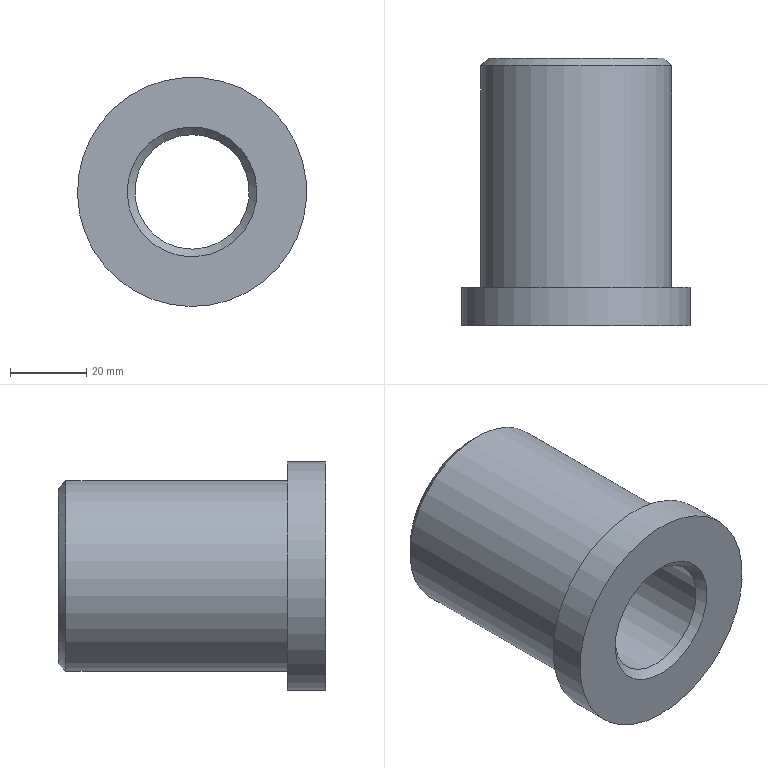Component | NX | SPINDLE_SLEEVE | 1 solid | 9 faces | box 60 x 70 x 60 mm | volume 95904 mm3 | plane 3 | cylinder 3 | cone 3 | commonest cylinder face diameters 30 x1 60 x1 50 x1
STEP:
#1=CARTESIAN_POINT('',(0.,0.,0.));
#2=DIRECTION('',(0.,0.,1.));
#3=DIRECTION('',(1.,0.,0.));
#4=AXIS2_PLACEMENT_3D('',#1,#2,#3);
#5=CARTESIAN_POINT('',(289.146,-15.,110.278));
#6=VERTEX_POINT('',#5);
#7=CARTESIAN_POINT('',(300.,-15.,90.));
#8=DIRECTION('',(0.,1.,0.));
#9=DIRECTION('',(-0.4719,0.,0.8817));
#10=AXIS2_PLACEMENT_3D('',#7,#8,#9);
#11=CIRCLE('',#10,23.);
#12=CARTESIAN_POINT('',(322.041,-15.,101.797));
#13=DIRECTION('',(0.,1.,0.));
#14=DIRECTION('',(-0.4719,0.,0.8817));
#15=AXIS2_PLACEMENT_3D('',#12,#13,#14);
#16=PLANE('',#15);
#17=CARTESIAN_POINT('',(-0.,-25.));
#18=DIRECTION('',(1.,0.));
#19=AXIS2_PLACEMENT_2D('',#17,#18);
#20=CIRCLE('',#19,23.);
#21=(GEOMETRIC_REPRESENTATION_CONTEXT(2)PARAMETRIC_REPRESENTATION_CONTEXT()REPRESENTATION_CONTEXT('',''));
#22=DEFINITIONAL_REPRESENTATION('',(#20),#21);
#23=PCURVE('',#16,#22);
#24=CARTESIAN_POINT('',(300.,-17.,90.));
#25=DIRECTION('',(0.,-1.,0.));
#26=DIRECTION('',(0.4719,0.,-0.8817));
#27=AXIS2_PLACEMENT_3D('',#24,#25,#26);
#28=CONICAL_SURFACE('',#27,25.,0.7854);
#29=CARTESIAN_POINT('',(9.425,-2.));
#30=DIRECTION('',(-1.,0.));
#31=VECTOR('',#30,1.);
#32=LINE('',#29,#31);
#33=(GEOMETRIC_REPRESENTATION_CONTEXT(2)PARAMETRIC_REPRESENTATION_CONTEXT()REPRESENTATION_CONTEXT('',''));
#34=DEFINITIONAL_REPRESENTATION('',(#32),#33);
#35=PCURVE('',#28,#34);
#36=SURFACE_CURVE('',#11,(#23,#35),.PCURVE_S1.);
#37=EDGE_CURVE('',#6,#6,#36,.T.);
#38=ORIENTED_EDGE('',*,*,#37,.T.);
#39=EDGE_LOOP('',(#38));
#40=FACE_BOUND('',#39,.T.);
#41=CARTESIAN_POINT('',(291.978,-15.,104.988));
#42=VERTEX_POINT('',#41);
#43=CARTESIAN_POINT('',(300.,-15.,90.));
#44=DIRECTION('',(0.,-1.,0.));
#45=DIRECTION('',(-0.4719,0.,0.8817));
#46=AXIS2_PLACEMENT_3D('',#43,#44,#45);
#47=CIRCLE('',#46,17.);
#48=CARTESIAN_POINT('',(17.,-25.));
#49=CARTESIAN_POINT('',(17.,-54.445));
#50=CARTESIAN_POINT('',(-8.5,-39.722));
#51=CARTESIAN_POINT('',(-34.,-25.));
#52=CARTESIAN_POINT('',(-8.5,-10.278));
#53=CARTESIAN_POINT('',(17.,4.445));
#54=CARTESIAN_POINT('',(17.,-25.));
#55=(BOUNDED_CURVE()B_SPLINE_CURVE(2,(#48,#49,#50,#51,#52,#53,#54),.UNSPECIFIED.,.T.,.F.)B_SPLINE_CURVE_WITH_KNOTS((1,2,2,2,2,1),(-2.094,0.,2.094,4.189,6.283,8.378),.UNSPECIFIED.)CURVE()GEOMETRIC_REPRESENTATION_ITEM()RATIONAL_B_SPLINE_CURVE((1.,0.5,1.,0.5,1.,0.5,1.))REPRESENTATION_ITEM(''));
#56=(GEOMETRIC_REPRESENTATION_CONTEXT(2)PARAMETRIC_REPRESENTATION_CONTEXT()REPRESENTATION_CONTEXT('',''));
#57=DEFINITIONAL_REPRESENTATION('',(#55),#56);
#58=PCURVE('',#16,#57);
#59=CARTESIAN_POINT('',(300.,-15.,90.));
#60=DIRECTION('',(0.,1.,0.));
#61=DIRECTION('',(-0.4719,0.,0.8817));
#62=AXIS2_PLACEMENT_3D('',#59,#60,#61);
#63=CONICAL_SURFACE('',#62,17.,0.7854);
#64=CARTESIAN_POINT('',(6.283,0.));
#65=DIRECTION('',(-1.,0.));
#66=VECTOR('',#65,1.);
#67=LINE('',#64,#66);
#68=(GEOMETRIC_REPRESENTATION_CONTEXT(2)PARAMETRIC_REPRESENTATION_CONTEXT()REPRESENTATION_CONTEXT('',''));
#69=DEFINITIONAL_REPRESENTATION('',(#67),#68);
#70=PCURVE('',#63,#69);
#71=SURFACE_CURVE('',#47,(#58,#70),.PCURVE_S1.);
#72=EDGE_CURVE('',#42,#42,#71,.T.);
#73=ORIENTED_EDGE('',*,*,#72,.T.);
#74=EDGE_LOOP('',(#73));
#75=FACE_BOUND('',#74,.T.);
#76=ADVANCED_FACE('',(#40,#75),#16,.T.);
#77=CARTESIAN_POINT('',(307.078,-17.,76.775));
#78=VERTEX_POINT('',#77);
#79=CARTESIAN_POINT('',(292.922,-17.,103.225));
#80=VERTEX_POINT('',#79);
#81=CARTESIAN_POINT('',(300.,-17.,90.));
#82=DIRECTION('',(0.,1.,0.));
#83=DIRECTION('',(-0.4719,0.,0.8817));
#84=AXIS2_PLACEMENT_3D('',#81,#82,#83);
#85=CIRCLE('',#84,15.);
#86=CARTESIAN_POINT('',(300.,-75.,90.));
#87=DIRECTION('',(0.,-1.,0.));
#88=DIRECTION('',(0.4719,0.,-0.8817));
#89=AXIS2_PLACEMENT_3D('',#86,#87,#88);
#90=CYLINDRICAL_SURFACE('',#89,15.);
#91=CARTESIAN_POINT('',(9.425,-58.));
#92=DIRECTION('',(-1.,0.));
#93=VECTOR('',#92,1.);
#94=LINE('',#91,#93);
#95=(GEOMETRIC_REPRESENTATION_CONTEXT(2)PARAMETRIC_REPRESENTATION_CONTEXT()REPRESENTATION_CONTEXT('',''));
#96=DEFINITIONAL_REPRESENTATION('',(#94),#95);
#97=PCURVE('',#90,#96);
#98=CARTESIAN_POINT('',(-0.,-2.));
#99=DIRECTION('',(1.,0.));
#100=VECTOR('',#99,1.);
#101=LINE('',#98,#100);
#102=(GEOMETRIC_REPRESENTATION_CONTEXT(2)PARAMETRIC_REPRESENTATION_CONTEXT()REPRESENTATION_CONTEXT('',''));
#103=DEFINITIONAL_REPRESENTATION('',(#101),#102);
#104=PCURVE('',#63,#103);
#105=SURFACE_CURVE('',#85,(#97,#104),.PCURVE_S1.);
#106=EDGE_CURVE('',#78,#80,#105,.T.);
#107=ORIENTED_EDGE('',*,*,#106,.F.);
#108=CARTESIAN_POINT('',(307.078,-83.,76.775));
#109=VERTEX_POINT('',#108);
#110=CARTESIAN_POINT('',(307.078,-17.,76.775));
#111=CARTESIAN_POINT('',(307.078,-83.,76.775));
#112=B_SPLINE_CURVE_WITH_KNOTS('',1,(#110,#111),.UNSPECIFIED.,.F.,.F.,(2,2),(-58.,8.),.PIECEWISE_BEZIER_KNOTS.);
#113=CARTESIAN_POINT('',(6.283,0.));
#114=DIRECTION('',(0.,1.));
#115=VECTOR('',#114,1.);
#116=LINE('',#113,#115);
#117=(GEOMETRIC_REPRESENTATION_CONTEXT(2)PARAMETRIC_REPRESENTATION_CONTEXT()REPRESENTATION_CONTEXT('',''));
#118=DEFINITIONAL_REPRESENTATION('',(#116),#117);
#119=PCURVE('',#90,#118);
#120=CARTESIAN_POINT('',(0.,0.));
#121=DIRECTION('',(0.,1.));
#122=VECTOR('',#121,1.);
#123=LINE('',#120,#122);
#124=(GEOMETRIC_REPRESENTATION_CONTEXT(2)PARAMETRIC_REPRESENTATION_CONTEXT()REPRESENTATION_CONTEXT('',''));
#125=DEFINITIONAL_REPRESENTATION('',(#123),#124);
#126=PCURVE('',#90,#125);
#127=SEAM_CURVE('',#112,(#119,#126),.PCURVE_S1.);
#128=EDGE_CURVE('',#78,#109,#127,.T.);
#129=ORIENTED_EDGE('',*,*,#128,.T.);
#130=CARTESIAN_POINT('',(300.,-83.,90.));
#131=DIRECTION('',(0.,-1.,0.));
#132=DIRECTION('',(0.4719,0.,-0.8817));
#133=AXIS2_PLACEMENT_3D('',#130,#131,#132);
#134=CIRCLE('',#133,15.);
#135=CARTESIAN_POINT('',(0.,8.));
#136=DIRECTION('',(1.,0.));
#137=VECTOR('',#136,1.);
#138=LINE('',#135,#137);
#139=(GEOMETRIC_REPRESENTATION_CONTEXT(2)PARAMETRIC_REPRESENTATION_CONTEXT()REPRESENTATION_CONTEXT('',''));
#140=DEFINITIONAL_REPRESENTATION('',(#138),#139);
#141=PCURVE('',#90,#140);
#142=CARTESIAN_POINT('',(300.,-83.,90.));
#143=DIRECTION('',(0.,-1.,0.));
#144=DIRECTION('',(0.4719,0.,-0.8817));
#145=AXIS2_PLACEMENT_3D('',#142,#143,#144);
#146=CONICAL_SURFACE('',#145,15.,0.7854);
#147=CARTESIAN_POINT('',(0.,0.));
#148=DIRECTION('',(1.,-0.));
#149=VECTOR('',#148,1.);
#150=LINE('',#147,#149);
#151=(GEOMETRIC_REPRESENTATION_CONTEXT(2)PARAMETRIC_REPRESENTATION_CONTEXT()REPRESENTATION_CONTEXT('',''));
#152=DEFINITIONAL_REPRESENTATION('',(#150),#151);
#153=PCURVE('',#146,#152);
#154=SURFACE_CURVE('',#134,(#141,#153),.PCURVE_S1.);
#155=EDGE_CURVE('',#109,#109,#154,.T.);
#156=ORIENTED_EDGE('',*,*,#155,.F.);
#157=ORIENTED_EDGE('',*,*,#128,.F.);
#158=CARTESIAN_POINT('',(300.,-17.,90.));
#159=DIRECTION('',(0.,1.,0.));
#160=DIRECTION('',(-0.4719,0.,0.8817));
#161=AXIS2_PLACEMENT_3D('',#158,#159,#160);
#162=CIRCLE('',#161,15.);
#163=CARTESIAN_POINT('',(3.142,-58.));
#164=DIRECTION('',(-1.,0.));
#165=VECTOR('',#164,1.);
#166=LINE('',#163,#165);
#167=(GEOMETRIC_REPRESENTATION_CONTEXT(2)PARAMETRIC_REPRESENTATION_CONTEXT()REPRESENTATION_CONTEXT('',''));
#168=DEFINITIONAL_REPRESENTATION('',(#166),#167);
#169=PCURVE('',#90,#168);
#170=CARTESIAN_POINT('',(0.,-2.));
#171=DIRECTION('',(1.,-0.));
#172=VECTOR('',#171,1.);
#173=LINE('',#170,#172);
#174=(GEOMETRIC_REPRESENTATION_CONTEXT(2)PARAMETRIC_REPRESENTATION_CONTEXT()REPRESENTATION_CONTEXT('',''));
#175=DEFINITIONAL_REPRESENTATION('',(#173),#174);
#176=PCURVE('',#63,#175);
#177=SURFACE_CURVE('',#162,(#169,#176),.PCURVE_S1.);
#178=EDGE_CURVE('',#80,#78,#177,.T.);
#179=ORIENTED_EDGE('',*,*,#178,.F.);
#180=EDGE_LOOP('',(#107,#129,#156,#157,#179));
#181=FACE_BOUND('',#180,.F.);
#182=ADVANCED_FACE('',(#181),#90,.F.);
#183=CARTESIAN_POINT('',(308.022,-85.,75.012));
#184=VERTEX_POINT('',#183);
#185=CARTESIAN_POINT('',(300.,-85.,90.));
#186=DIRECTION('',(0.,1.,0.));
#187=DIRECTION('',(0.4719,0.,-0.8817));
#188=AXIS2_PLACEMENT_3D('',#185,#186,#187);
#189=CIRCLE('',#188,17.);
#190=CARTESIAN_POINT('',(313.225,-85.,97.078));
#191=DIRECTION('',(0.,-1.,0.));
#192=DIRECTION('',(0.4719,0.,-0.8817));
#193=AXIS2_PLACEMENT_3D('',#190,#191,#192);
#194=PLANE('',#193);
#195=CARTESIAN_POINT('',(17.,-15.));
#196=CARTESIAN_POINT('',(17.,-44.445));
#197=CARTESIAN_POINT('',(-8.5,-29.722));
#198=CARTESIAN_POINT('',(-34.,-15.));
#199=CARTESIAN_POINT('',(-8.5,-0.2776));
#200=CARTESIAN_POINT('',(17.,14.445));
#201=CARTESIAN_POINT('',(17.,-15.));
#202=(BOUNDED_CURVE()B_SPLINE_CURVE(2,(#195,#196,#197,#198,#199,#200,#201),.UNSPECIFIED.,.T.,.F.)B_SPLINE_CURVE_WITH_KNOTS((1,2,2,2,2,1),(-2.094,0.,2.094,4.189,6.283,8.378),.UNSPECIFIED.)CURVE()GEOMETRIC_REPRESENTATION_ITEM()RATIONAL_B_SPLINE_CURVE((1.,0.5,1.,0.5,1.,0.5,1.))REPRESENTATION_ITEM(''));
#203=(GEOMETRIC_REPRESENTATION_CONTEXT(2)PARAMETRIC_REPRESENTATION_CONTEXT()REPRESENTATION_CONTEXT('',''));
#204=DEFINITIONAL_REPRESENTATION('',(#202),#203);
#205=PCURVE('',#194,#204);
#206=CARTESIAN_POINT('',(6.283,2.));
#207=DIRECTION('',(-1.,0.));
#208=VECTOR('',#207,1.);
#209=LINE('',#206,#208);
#210=(GEOMETRIC_REPRESENTATION_CONTEXT(2)PARAMETRIC_REPRESENTATION_CONTEXT()REPRESENTATION_CONTEXT('',''));
#211=DEFINITIONAL_REPRESENTATION('',(#209),#210);
#212=PCURVE('',#146,#211);
#213=SURFACE_CURVE('',#189,(#205,#212),.PCURVE_S1.);
#214=EDGE_CURVE('',#184,#184,#213,.T.);
#215=ORIENTED_EDGE('',*,*,#214,.T.);
#216=EDGE_LOOP('',(#215));
#217=FACE_BOUND('',#216,.T.);
#218=CARTESIAN_POINT('',(314.157,-85.,63.55));
#219=VERTEX_POINT('',#218);
#220=CARTESIAN_POINT('',(300.,-85.,90.));
#221=DIRECTION('',(0.,-1.,0.));
#222=DIRECTION('',(0.4719,0.,-0.8817));
#223=AXIS2_PLACEMENT_3D('',#220,#221,#222);
#224=CIRCLE('',#223,30.);
#225=CARTESIAN_POINT('',(0.,-15.));
#226=DIRECTION('',(1.,0.));
#227=AXIS2_PLACEMENT_2D('',#225,#226);
#228=CIRCLE('',#227,30.);
#229=(GEOMETRIC_REPRESENTATION_CONTEXT(2)PARAMETRIC_REPRESENTATION_CONTEXT()REPRESENTATION_CONTEXT('',''));
#230=DEFINITIONAL_REPRESENTATION('',(#228),#229);
#231=PCURVE('',#194,#230);
#232=CARTESIAN_POINT('',(300.,-75.,90.));
#233=DIRECTION('',(0.,-1.,0.));
#234=DIRECTION('',(0.4719,0.,-0.8817));
#235=AXIS2_PLACEMENT_3D('',#232,#233,#234);
#236=CYLINDRICAL_SURFACE('',#235,30.);
#237=CARTESIAN_POINT('',(0.,10.));
#238=DIRECTION('',(1.,0.));
#239=VECTOR('',#238,1.);
#240=LINE('',#237,#239);
#241=(GEOMETRIC_REPRESENTATION_CONTEXT(2)PARAMETRIC_REPRESENTATION_CONTEXT()REPRESENTATION_CONTEXT('',''));
#242=DEFINITIONAL_REPRESENTATION('',(#240),#241);
#243=PCURVE('',#236,#242);
#244=SURFACE_CURVE('',#224,(#231,#243),.PCURVE_S1.);
#245=EDGE_CURVE('',#219,#219,#244,.T.);
#246=ORIENTED_EDGE('',*,*,#245,.T.);
#247=EDGE_LOOP('',(#246));
#248=FACE_BOUND('',#247,.T.);
#249=ADVANCED_FACE('',(#217,#248),#194,.T.);
#250=CARTESIAN_POINT('',(314.157,-75.,63.55));
#251=VERTEX_POINT('',#250);
#252=CARTESIAN_POINT('',(300.,-75.,90.));
#253=DIRECTION('',(0.,-1.,0.));
#254=DIRECTION('',(0.4719,0.,-0.8817));
#255=AXIS2_PLACEMENT_3D('',#252,#253,#254);
#256=CIRCLE('',#255,30.);
#257=CARTESIAN_POINT('',(0.,0.));
#258=DIRECTION('',(1.,0.));
#259=VECTOR('',#258,1.);
#260=LINE('',#257,#259);
#261=(GEOMETRIC_REPRESENTATION_CONTEXT(2)PARAMETRIC_REPRESENTATION_CONTEXT()REPRESENTATION_CONTEXT('',''));
#262=DEFINITIONAL_REPRESENTATION('',(#260),#261);
#263=PCURVE('',#236,#262);
#264=CARTESIAN_POINT('',(326.45,-75.,104.157));
#265=DIRECTION('',(0.,1.,0.));
#266=DIRECTION('',(-0.4719,0.,0.8817));
#267=AXIS2_PLACEMENT_3D('',#264,#265,#266);
#268=PLANE('',#267);
#269=CARTESIAN_POINT('',(-30.,-30.));
#270=CARTESIAN_POINT('',(-30.,21.962));
#271=CARTESIAN_POINT('',(15.,-4.019));
#272=CARTESIAN_POINT('',(60.,-30.));
#273=CARTESIAN_POINT('',(15.,-55.981));
#274=CARTESIAN_POINT('',(-30.,-81.962));
#275=CARTESIAN_POINT('',(-30.,-30.));
#276=(BOUNDED_CURVE()B_SPLINE_CURVE(2,(#269,#270,#271,#272,#273,#274,#275),.UNSPECIFIED.,.T.,.F.)B_SPLINE_CURVE_WITH_KNOTS((1,2,2,2,2,1),(-2.094,0.,2.094,4.189,6.283,8.378),.UNSPECIFIED.)CURVE()GEOMETRIC_REPRESENTATION_ITEM()RATIONAL_B_SPLINE_CURVE((1.,0.5,1.,0.5,1.,0.5,1.))REPRESENTATION_ITEM(''));
#277=(GEOMETRIC_REPRESENTATION_CONTEXT(2)PARAMETRIC_REPRESENTATION_CONTEXT()REPRESENTATION_CONTEXT('',''));
#278=DEFINITIONAL_REPRESENTATION('',(#276),#277);
#279=PCURVE('',#268,#278);
#280=SURFACE_CURVE('',#256,(#263,#279),.PCURVE_S1.);
#281=EDGE_CURVE('',#251,#251,#280,.T.);
#282=ORIENTED_EDGE('',*,*,#281,.T.);
#283=CARTESIAN_POINT('',(314.157,-75.,63.55));
#284=CARTESIAN_POINT('',(314.157,-85.,63.55));
#285=B_SPLINE_CURVE_WITH_KNOTS('',1,(#283,#284),.UNSPECIFIED.,.F.,.F.,(2,2),(0.,10.),.PIECEWISE_BEZIER_KNOTS.);
#286=CARTESIAN_POINT('',(6.283,0.));
#287=DIRECTION('',(0.,1.));
#288=VECTOR('',#287,1.);
#289=LINE('',#286,#288);
#290=(GEOMETRIC_REPRESENTATION_CONTEXT(2)PARAMETRIC_REPRESENTATION_CONTEXT()REPRESENTATION_CONTEXT('',''));
#291=DEFINITIONAL_REPRESENTATION('',(#289),#290);
#292=PCURVE('',#236,#291);
#293=CARTESIAN_POINT('',(0.,0.));
#294=DIRECTION('',(0.,1.));
#295=VECTOR('',#294,1.);
#296=LINE('',#293,#295);
#297=(GEOMETRIC_REPRESENTATION_CONTEXT(2)PARAMETRIC_REPRESENTATION_CONTEXT()REPRESENTATION_CONTEXT('',''));
#298=DEFINITIONAL_REPRESENTATION('',(#296),#297);
#299=PCURVE('',#236,#298);
#300=SEAM_CURVE('',#285,(#292,#299),.PCURVE_S1.);
#301=EDGE_CURVE('',#251,#219,#300,.T.);
#302=ORIENTED_EDGE('',*,*,#301,.T.);
#303=ORIENTED_EDGE('',*,*,#245,.F.);
#304=ORIENTED_EDGE('',*,*,#301,.F.);
#305=EDGE_LOOP('',(#282,#302,#303,#304));
#306=FACE_BOUND('',#305,.T.);
#307=ADVANCED_FACE('',(#306),#236,.T.);
#308=CARTESIAN_POINT('',(311.797,-75.,67.959));
#309=VERTEX_POINT('',#308);
#310=CARTESIAN_POINT('',(300.,-75.,90.));
#311=DIRECTION('',(0.,-1.,0.));
#312=DIRECTION('',(0.4719,0.,-0.8817));
#313=AXIS2_PLACEMENT_3D('',#310,#311,#312);
#314=CIRCLE('',#313,25.);
#315=CARTESIAN_POINT('',(-25.,-30.));
#316=CARTESIAN_POINT('',(-25.,13.301));
#317=CARTESIAN_POINT('',(12.5,-8.349));
#318=CARTESIAN_POINT('',(50.,-30.));
#319=CARTESIAN_POINT('',(12.5,-51.651));
#320=CARTESIAN_POINT('',(-25.,-73.301));
#321=CARTESIAN_POINT('',(-25.,-30.));
#322=(BOUNDED_CURVE()B_SPLINE_CURVE(2,(#315,#316,#317,#318,#319,#320,#321),.UNSPECIFIED.,.T.,.F.)B_SPLINE_CURVE_WITH_KNOTS((1,2,2,2,2,1),(-2.094,0.,2.094,4.189,6.283,8.378),.UNSPECIFIED.)CURVE()GEOMETRIC_REPRESENTATION_ITEM()RATIONAL_B_SPLINE_CURVE((1.,0.5,1.,0.5,1.,0.5,1.))REPRESENTATION_ITEM(''));
#323=(GEOMETRIC_REPRESENTATION_CONTEXT(2)PARAMETRIC_REPRESENTATION_CONTEXT()REPRESENTATION_CONTEXT('',''));
#324=DEFINITIONAL_REPRESENTATION('',(#322),#323);
#325=PCURVE('',#268,#324);
#326=CARTESIAN_POINT('',(300.,-75.,90.));
#327=DIRECTION('',(0.,-1.,0.));
#328=DIRECTION('',(0.4719,0.,-0.8817));
#329=AXIS2_PLACEMENT_3D('',#326,#327,#328);
#330=CYLINDRICAL_SURFACE('',#329,25.);
#331=CARTESIAN_POINT('',(0.,0.));
#332=DIRECTION('',(1.,0.));
#333=VECTOR('',#332,1.);
#334=LINE('',#331,#333);
#335=(GEOMETRIC_REPRESENTATION_CONTEXT(2)PARAMETRIC_REPRESENTATION_CONTEXT()REPRESENTATION_CONTEXT('',''));
#336=DEFINITIONAL_REPRESENTATION('',(#334),#335);
#337=PCURVE('',#330,#336);
#338=SURFACE_CURVE('',#314,(#325,#337),.PCURVE_S1.);
#339=EDGE_CURVE('',#309,#309,#338,.T.);
#340=ORIENTED_EDGE('',*,*,#339,.T.);
#341=EDGE_LOOP('',(#340));
#342=FACE_BOUND('',#341,.T.);
#343=ORIENTED_EDGE('',*,*,#281,.F.);
#344=EDGE_LOOP('',(#343));
#345=FACE_BOUND('',#344,.T.);
#346=ADVANCED_FACE('',(#342,#345),#268,.T.);
#347=CARTESIAN_POINT('',(288.203,-17.,112.041));
#348=VERTEX_POINT('',#347);
#349=CARTESIAN_POINT('',(311.797,-17.,67.959));
#350=VERTEX_POINT('',#349);
#351=CARTESIAN_POINT('',(300.,-17.,90.));
#352=DIRECTION('',(0.,-1.,0.));
#353=DIRECTION('',(-0.4719,0.,0.8817));
#354=AXIS2_PLACEMENT_3D('',#351,#352,#353);
#355=CIRCLE('',#354,25.);
#356=CARTESIAN_POINT('',(3.142,-58.));
#357=DIRECTION('',(1.,0.));
#358=VECTOR('',#357,1.);
#359=LINE('',#356,#358);
#360=(GEOMETRIC_REPRESENTATION_CONTEXT(2)PARAMETRIC_REPRESENTATION_CONTEXT()REPRESENTATION_CONTEXT('',''));
#361=DEFINITIONAL_REPRESENTATION('',(#359),#360);
#362=PCURVE('',#330,#361);
#363=CARTESIAN_POINT('',(3.142,0.));
#364=DIRECTION('',(1.,-0.));
#365=VECTOR('',#364,1.);
#366=LINE('',#363,#365);
#367=(GEOMETRIC_REPRESENTATION_CONTEXT(2)PARAMETRIC_REPRESENTATION_CONTEXT()REPRESENTATION_CONTEXT('',''));
#368=DEFINITIONAL_REPRESENTATION('',(#366),#367);
#369=PCURVE('',#28,#368);
#370=SURFACE_CURVE('',#355,(#362,#369),.PCURVE_S1.);
#371=EDGE_CURVE('',#348,#350,#370,.T.);
#372=ORIENTED_EDGE('',*,*,#371,.T.);
#373=CARTESIAN_POINT('',(311.797,-17.,67.959));
#374=CARTESIAN_POINT('',(311.797,-75.,67.959));
#375=B_SPLINE_CURVE_WITH_KNOTS('',1,(#373,#374),.UNSPECIFIED.,.F.,.F.,(2,2),(-58.,0.),.PIECEWISE_BEZIER_KNOTS.);
#376=CARTESIAN_POINT('',(6.283,0.));
#377=DIRECTION('',(0.,1.));
#378=VECTOR('',#377,1.);
#379=LINE('',#376,#378);
#380=(GEOMETRIC_REPRESENTATION_CONTEXT(2)PARAMETRIC_REPRESENTATION_CONTEXT()REPRESENTATION_CONTEXT('',''));
#381=DEFINITIONAL_REPRESENTATION('',(#379),#380);
#382=PCURVE('',#330,#381);
#383=CARTESIAN_POINT('',(0.,0.));
#384=DIRECTION('',(0.,1.));
#385=VECTOR('',#384,1.);
#386=LINE('',#383,#385);
#387=(GEOMETRIC_REPRESENTATION_CONTEXT(2)PARAMETRIC_REPRESENTATION_CONTEXT()REPRESENTATION_CONTEXT('',''));
#388=DEFINITIONAL_REPRESENTATION('',(#386),#387);
#389=PCURVE('',#330,#388);
#390=SEAM_CURVE('',#375,(#382,#389),.PCURVE_S1.);
#391=EDGE_CURVE('',#350,#309,#390,.T.);
#392=ORIENTED_EDGE('',*,*,#391,.T.);
#393=ORIENTED_EDGE('',*,*,#339,.F.);
#394=ORIENTED_EDGE('',*,*,#391,.F.);
#395=CARTESIAN_POINT('',(300.,-17.,90.));
#396=DIRECTION('',(0.,-1.,0.));
#397=DIRECTION('',(-0.4719,0.,0.8817));
#398=AXIS2_PLACEMENT_3D('',#395,#396,#397);
#399=CIRCLE('',#398,25.);
#400=CARTESIAN_POINT('',(-3.142,-58.));
#401=DIRECTION('',(1.,0.));
#402=VECTOR('',#401,1.);
#403=LINE('',#400,#402);
#404=(GEOMETRIC_REPRESENTATION_CONTEXT(2)PARAMETRIC_REPRESENTATION_CONTEXT()REPRESENTATION_CONTEXT('',''));
#405=DEFINITIONAL_REPRESENTATION('',(#403),#404);
#406=PCURVE('',#330,#405);
#407=CARTESIAN_POINT('',(3.142,-0.));
#408=DIRECTION('',(1.,0.));
#409=VECTOR('',#408,1.);
#410=LINE('',#407,#409);
#411=(GEOMETRIC_REPRESENTATION_CONTEXT(2)PARAMETRIC_REPRESENTATION_CONTEXT()REPRESENTATION_CONTEXT('',''));
#412=DEFINITIONAL_REPRESENTATION('',(#410),#411);
#413=PCURVE('',#28,#412);
#414=SURFACE_CURVE('',#399,(#406,#413),.PCURVE_S1.);
#415=EDGE_CURVE('',#350,#348,#414,.T.);
#416=ORIENTED_EDGE('',*,*,#415,.T.);
#417=EDGE_LOOP('',(#372,#392,#393,#394,#416));
#418=FACE_BOUND('',#417,.T.);
#419=ADVANCED_FACE('',(#418),#330,.T.);
#420=ORIENTED_EDGE('',*,*,#37,.F.);
#421=CARTESIAN_POINT('',(289.146,-15.,110.278));
#422=CARTESIAN_POINT('',(288.203,-17.,112.041));
#423=B_SPLINE_CURVE_WITH_KNOTS('',1,(#421,#422),.UNSPECIFIED.,.F.,.F.,(2,2),(-2.828,0.),.PIECEWISE_BEZIER_KNOTS.);
#424=CARTESIAN_POINT('',(9.425,0.));
#425=DIRECTION('',(0.,1.));
#426=VECTOR('',#425,1.);
#427=LINE('',#424,#426);
#428=(GEOMETRIC_REPRESENTATION_CONTEXT(2)PARAMETRIC_REPRESENTATION_CONTEXT()REPRESENTATION_CONTEXT('',''));
#429=DEFINITIONAL_REPRESENTATION('',(#427),#428);
#430=PCURVE('',#28,#429);
#431=CARTESIAN_POINT('',(3.142,0.));
#432=DIRECTION('',(0.,1.));
#433=VECTOR('',#432,1.);
#434=LINE('',#431,#433);
#435=(GEOMETRIC_REPRESENTATION_CONTEXT(2)PARAMETRIC_REPRESENTATION_CONTEXT()REPRESENTATION_CONTEXT('',''));
#436=DEFINITIONAL_REPRESENTATION('',(#434),#435);
#437=PCURVE('',#28,#436);
#438=SEAM_CURVE('',#423,(#430,#437),.PCURVE_S1.);
#439=EDGE_CURVE('',#6,#348,#438,.T.);
#440=ORIENTED_EDGE('',*,*,#439,.T.);
#441=ORIENTED_EDGE('',*,*,#415,.F.);
#442=ORIENTED_EDGE('',*,*,#371,.F.);
#443=ORIENTED_EDGE('',*,*,#439,.F.);
#444=EDGE_LOOP('',(#420,#440,#441,#442,#443));
#445=FACE_BOUND('',#444,.T.);
#446=ADVANCED_FACE('',(#445),#28,.T.);
#447=ORIENTED_EDGE('',*,*,#106,.T.);
#448=CARTESIAN_POINT('',(292.922,-17.,103.225));
#449=CARTESIAN_POINT('',(291.978,-15.,104.988));
#450=B_SPLINE_CURVE_WITH_KNOTS('',1,(#448,#449),.UNSPECIFIED.,.F.,.F.,(2,2),(-2.828,0.),.PIECEWISE_BEZIER_KNOTS.);
#451=CARTESIAN_POINT('',(6.283,0.));
#452=DIRECTION('',(0.,1.));
#453=VECTOR('',#452,1.);
#454=LINE('',#451,#453);
#455=(GEOMETRIC_REPRESENTATION_CONTEXT(2)PARAMETRIC_REPRESENTATION_CONTEXT()REPRESENTATION_CONTEXT('',''));
#456=DEFINITIONAL_REPRESENTATION('',(#454),#455);
#457=PCURVE('',#63,#456);
#458=CARTESIAN_POINT('',(-0.,0.));
#459=DIRECTION('',(0.,1.));
#460=VECTOR('',#459,1.);
#461=LINE('',#458,#460);
#462=(GEOMETRIC_REPRESENTATION_CONTEXT(2)PARAMETRIC_REPRESENTATION_CONTEXT()REPRESENTATION_CONTEXT('',''));
#463=DEFINITIONAL_REPRESENTATION('',(#461),#462);
#464=PCURVE('',#63,#463);
#465=SEAM_CURVE('',#450,(#457,#464),.PCURVE_S1.);
#466=EDGE_CURVE('',#80,#42,#465,.T.);
#467=ORIENTED_EDGE('',*,*,#466,.T.);
#468=ORIENTED_EDGE('',*,*,#72,.T.);
#469=ORIENTED_EDGE('',*,*,#466,.F.);
#470=ORIENTED_EDGE('',*,*,#178,.T.);
#471=EDGE_LOOP('',(#447,#467,#468,#469,#470));
#472=FACE_BOUND('',#471,.F.);
#473=ADVANCED_FACE('',(#472),#63,.F.);
#474=ORIENTED_EDGE('',*,*,#214,.T.);
#475=CARTESIAN_POINT('',(307.078,-83.,76.775));
#476=CARTESIAN_POINT('',(308.022,-85.,75.012));
#477=B_SPLINE_CURVE_WITH_KNOTS('',1,(#475,#476),.UNSPECIFIED.,.F.,.F.,(2,2),(0.,2.828),.PIECEWISE_BEZIER_KNOTS.);
#478=CARTESIAN_POINT('',(0.,0.));
#479=DIRECTION('',(0.,1.));
#480=VECTOR('',#479,1.);
#481=LINE('',#478,#480);
#482=(GEOMETRIC_REPRESENTATION_CONTEXT(2)PARAMETRIC_REPRESENTATION_CONTEXT()REPRESENTATION_CONTEXT('',''));
#483=DEFINITIONAL_REPRESENTATION('',(#481),#482);
#484=PCURVE('',#146,#483);
#485=CARTESIAN_POINT('',(6.283,0.));
#486=DIRECTION('',(0.,1.));
#487=VECTOR('',#486,1.);
#488=LINE('',#485,#487);
#489=(GEOMETRIC_REPRESENTATION_CONTEXT(2)PARAMETRIC_REPRESENTATION_CONTEXT()REPRESENTATION_CONTEXT('',''));
#490=DEFINITIONAL_REPRESENTATION('',(#488),#489);
#491=PCURVE('',#146,#490);
#492=SEAM_CURVE('',#477,(#484,#491),.PCURVE_S1.);
#493=EDGE_CURVE('',#109,#184,#492,.T.);
#494=ORIENTED_EDGE('',*,*,#493,.F.);
#495=ORIENTED_EDGE('',*,*,#155,.T.);
#496=ORIENTED_EDGE('',*,*,#493,.T.);
#497=EDGE_LOOP('',(#474,#494,#495,#496));
#498=FACE_BOUND('',#497,.F.);
#499=ADVANCED_FACE('',(#498),#146,.F.);
#500=CLOSED_SHELL('',(#76,#182,#249,#307,#346,#419,#446,#473,#499));
#501=MANIFOLD_SOLID_BREP('',#500);
#502=(LENGTH_UNIT()NAMED_UNIT(*)SI_UNIT(.MILLI.,.METRE.));
#503=UNCERTAINTY_MEASURE_WITH_UNIT(LENGTH_MEASURE(0.00001),#502,'','');
#504=(NAMED_UNIT(*)PLANE_ANGLE_UNIT()SI_UNIT($,.RADIAN.));
#505=(NAMED_UNIT(*)SI_UNIT($,.STERADIAN.)SOLID_ANGLE_UNIT());
#506=(GEOMETRIC_REPRESENTATION_CONTEXT(3)GLOBAL_UNCERTAINTY_ASSIGNED_CONTEXT((#503))GLOBAL_UNIT_ASSIGNED_CONTEXT((#502,#504,#505))REPRESENTATION_CONTEXT('',''));
#507=ADVANCED_BREP_SHAPE_REPRESENTATION('',(#4,#501),#506);